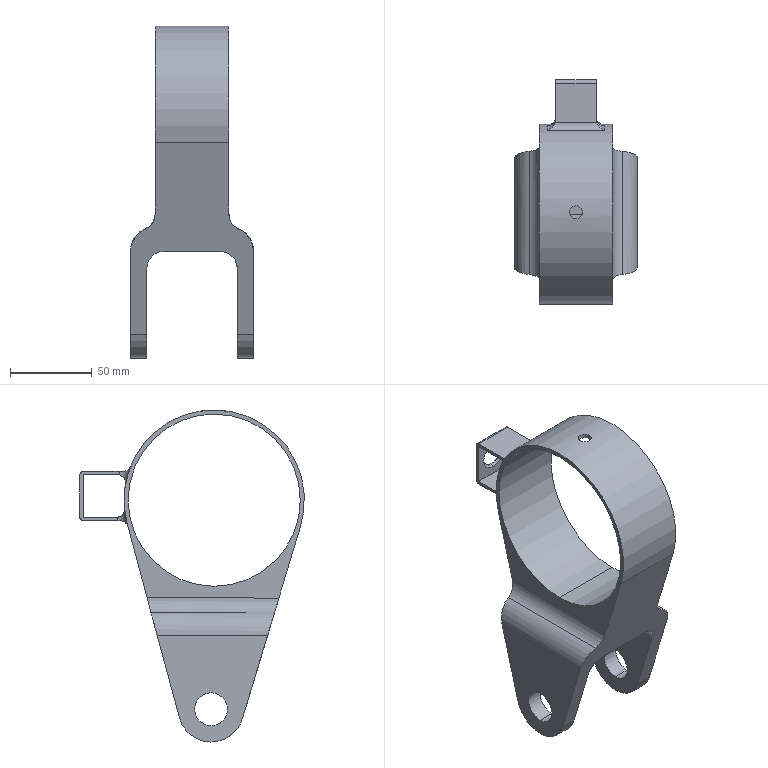Component | SolidWorks | dudukan2-1 | 1 solid | 54 faces | volume 249562 mm3 | cylinder 31 | plane 17 | torus 4 | cone 2 | commonest cylinder face diameters 20 x8 10 x7 40 x4 4 x3 8 x2 14 x2 105 x2 30 x2 | material ASTM A36 Steel